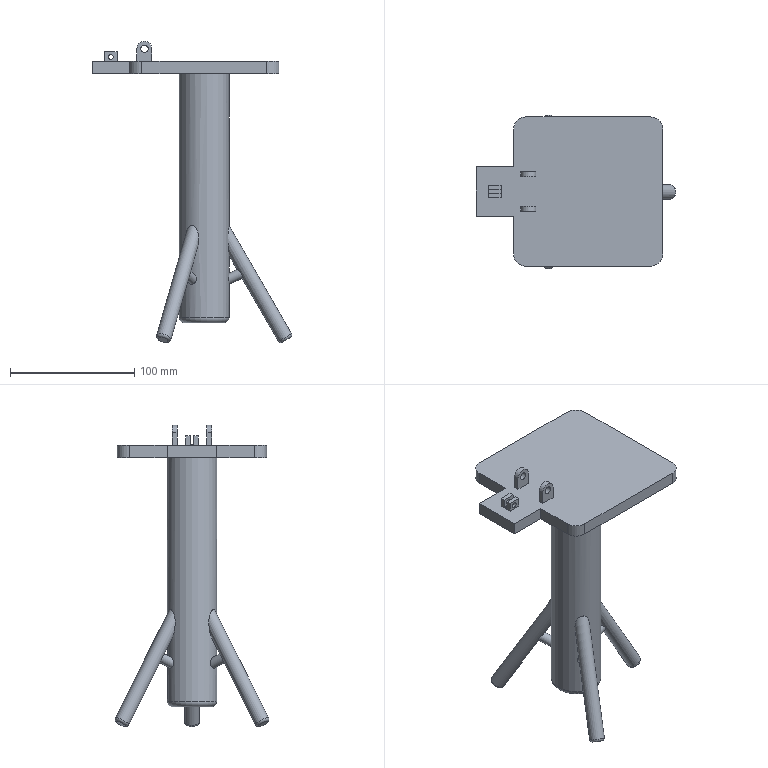Component | NX | SHEJI-WAIGUAN-2 | 1 solid | 52 faces | volume 440466 mm3 | plane 31 | cylinder 17 | torus 4 | commonest cylinder face diameters 12 x5 20 x4 8 x3 4 x2 6 x2 40 x1